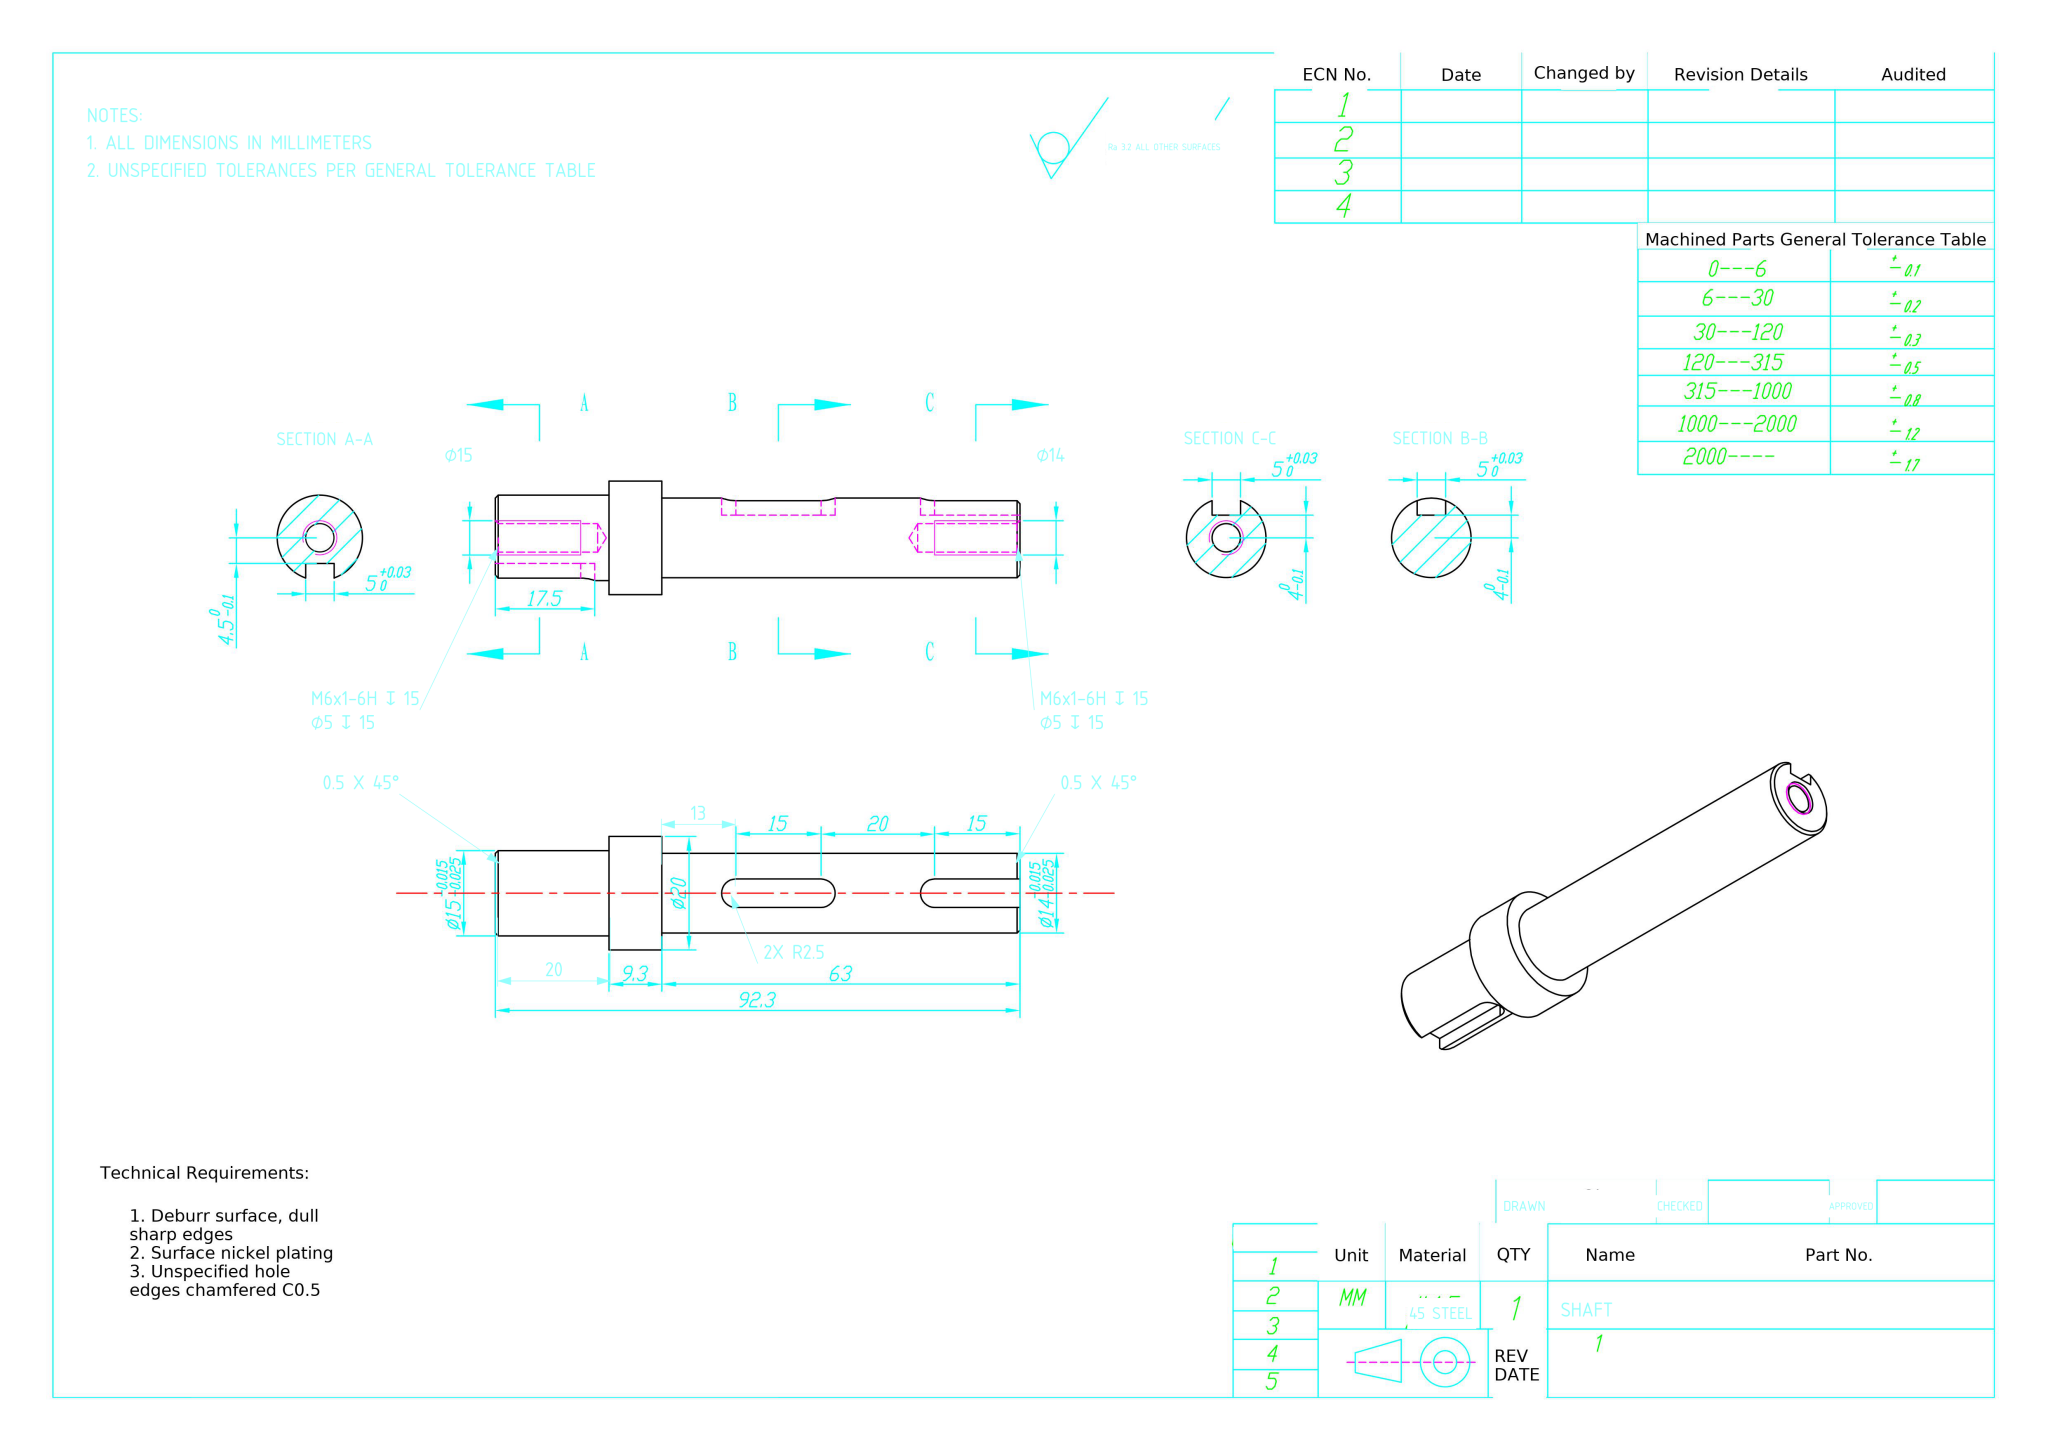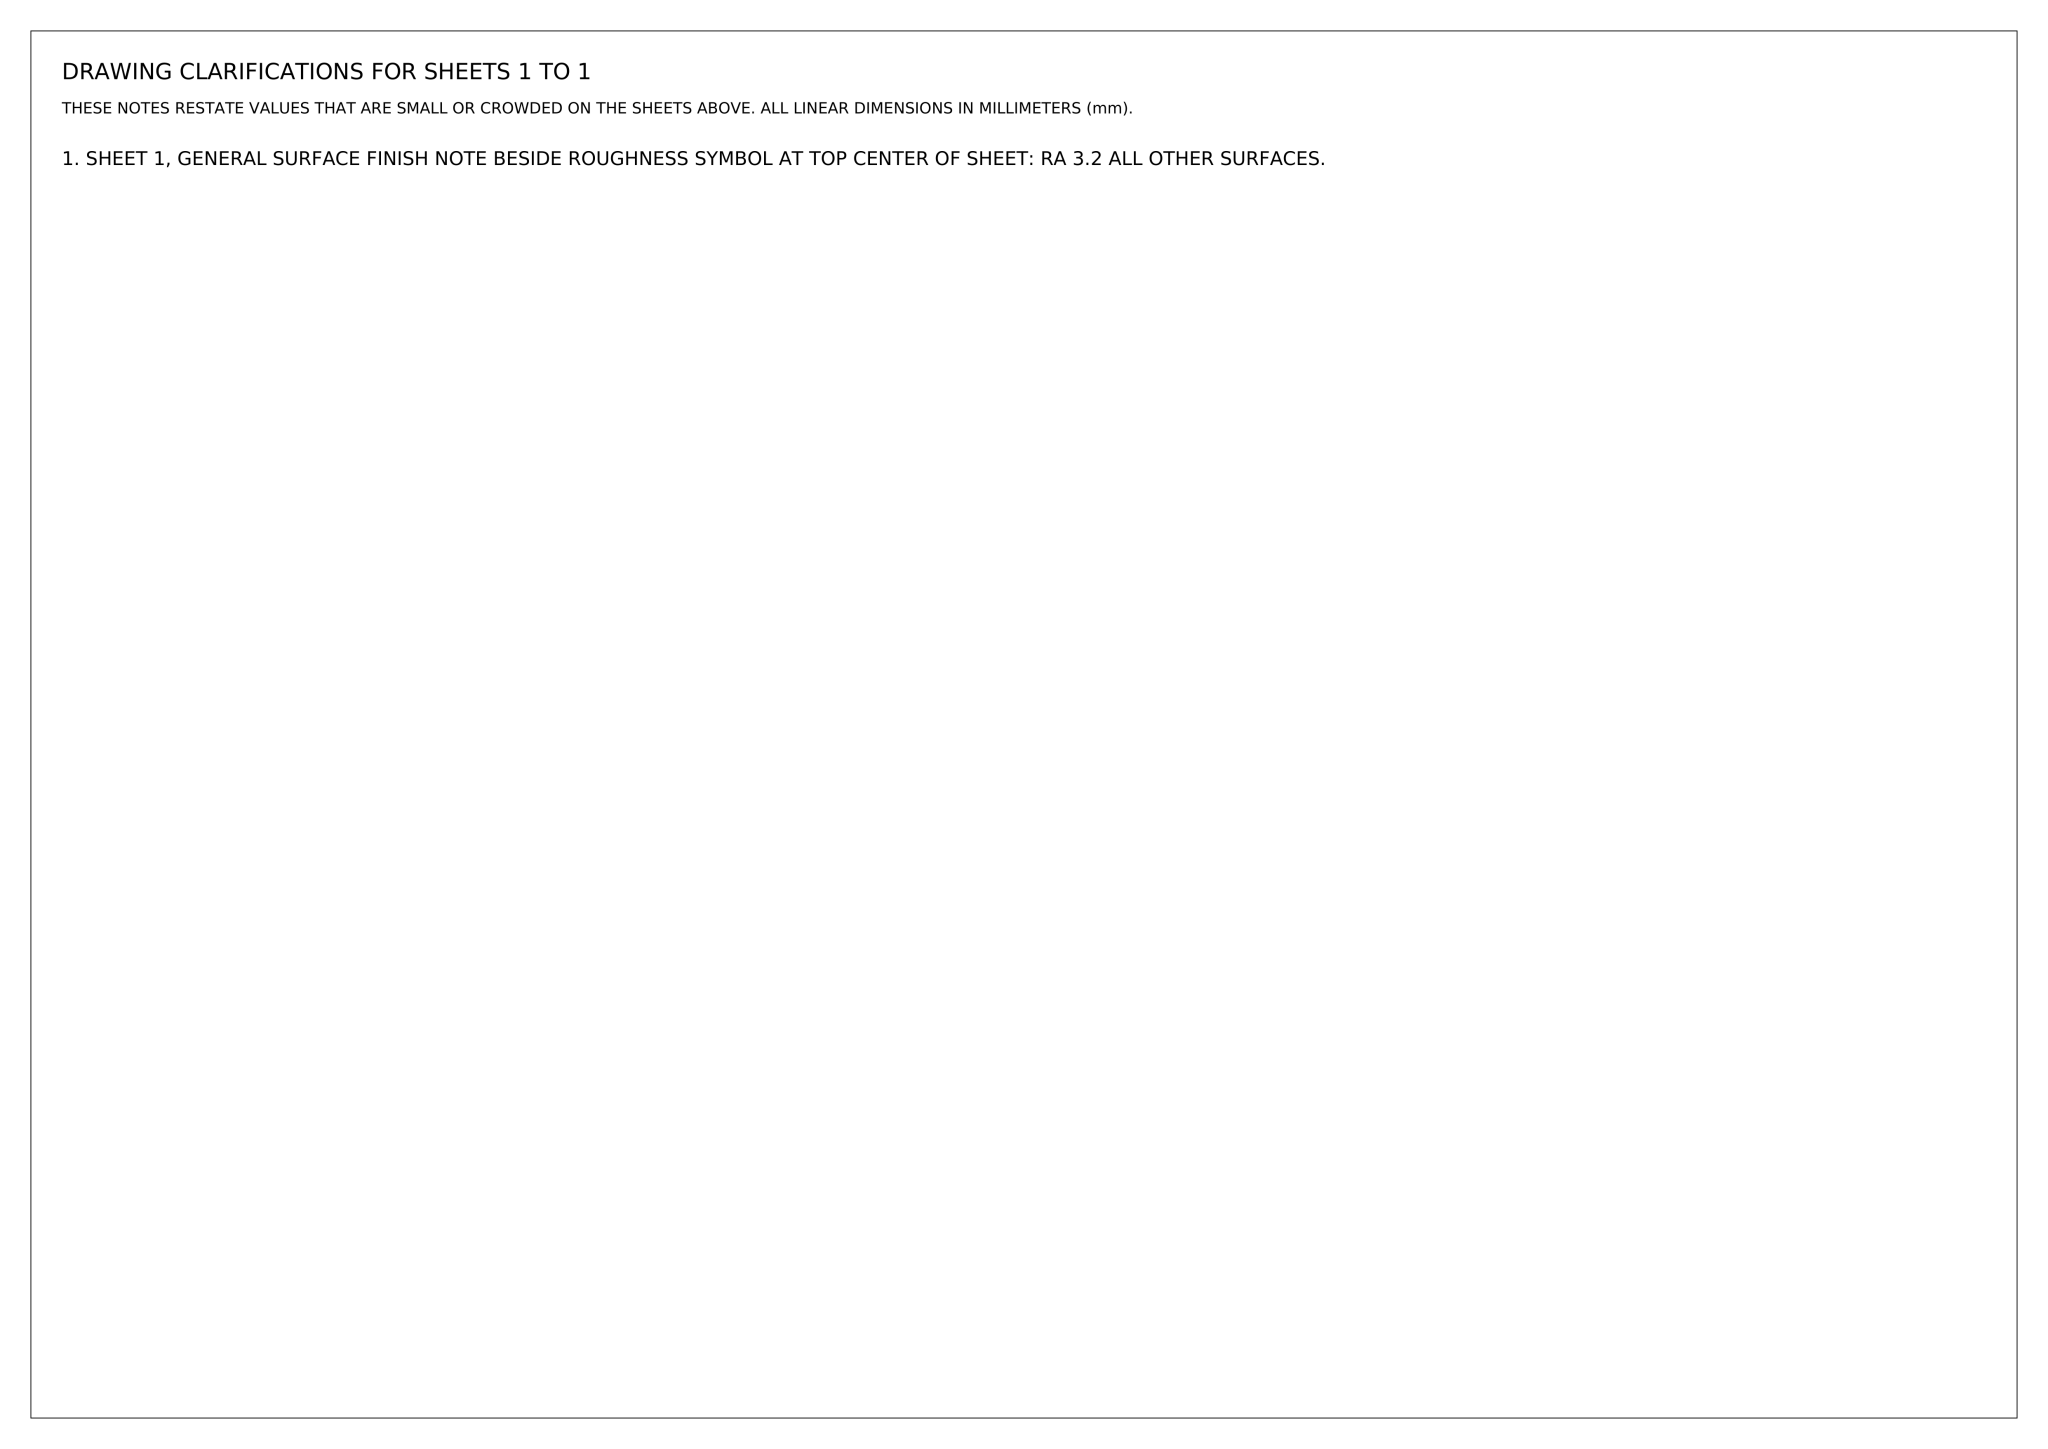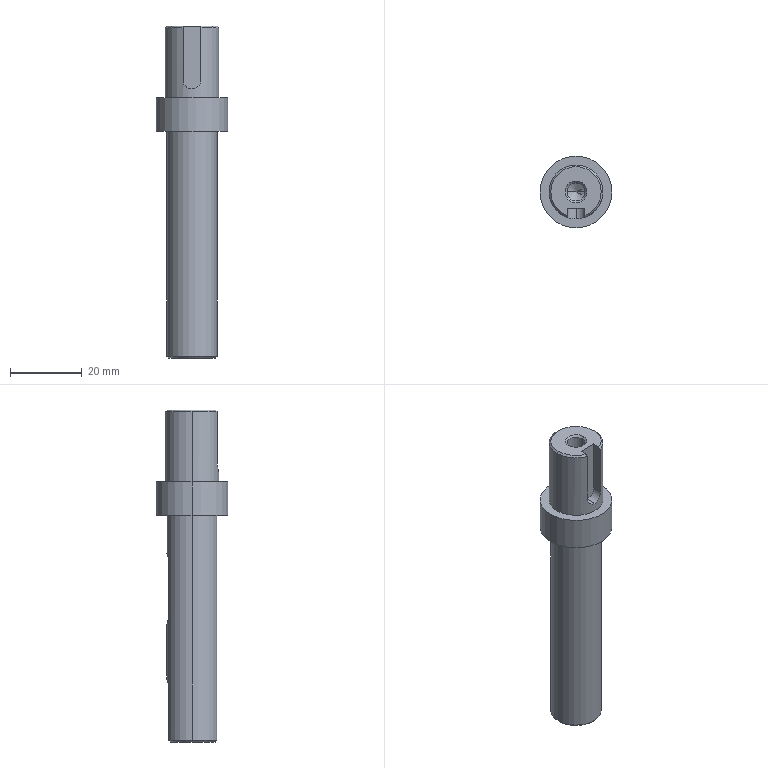Part | NX | mm | 1 solid | 44 faces | box 20 x 20 x 92.3 mm | volume 14658 mm3 | cylinder 17 | cone 14 | plane 13 | commonest cylinder face diameters 5 x11 20 x2 14 x2 15 x2